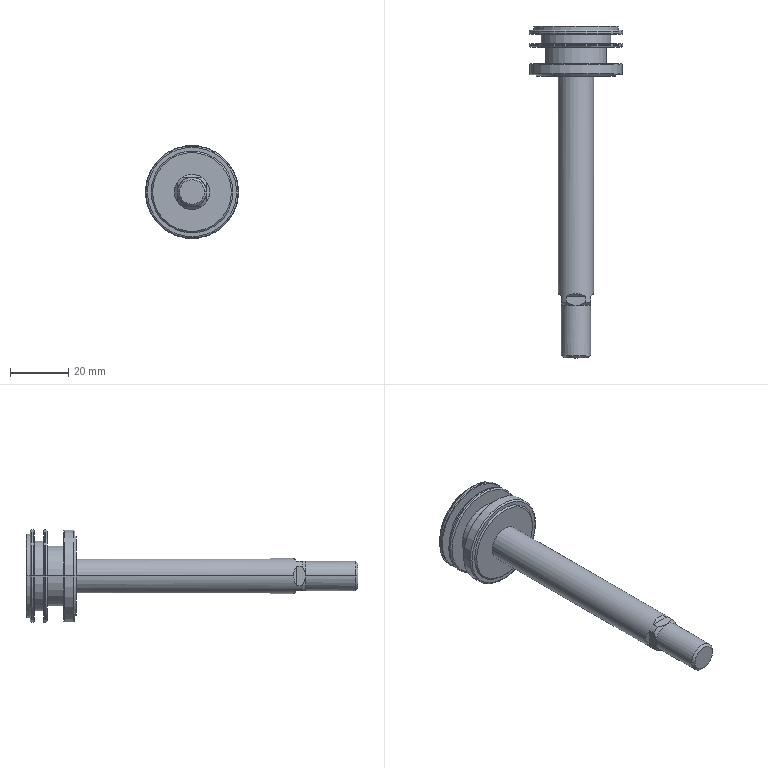Component | SolidWorks | SDAS_32x60_B_0-1_SDAS_32x60_B60_r-1 | 1 solid | 55 faces | box 31.9 x 113.5 x 31.9 mm | volume 19815 mm3 | plane 17 | cylinder 16 | cone 12 | torus 10 | commonest cylinder face diameters 31.9 x4 10 x2 28.9 x2 23.9 x2 20.8 x2 31.6 x2 12 x2
build123d program:
from build123d import *

# Parameters (mm, degrees)
CUT_EXTRUDE1_DEPTH      = 10
CUT_EXTRUDE1_DEPTH_BACK = 10
CUT_EXTRUDE2_DEPTH      = 10
CUT_EXTRUDE2_DEPTH_BACK = 10


with BuildPart() as part:
    # Sketch1 → Revolve1 (revolve)
    with BuildSketch(Plane.XY, mode=Mode.PRIVATE) as revolve1_sk:
        with BuildLine():
            Line((0, 0), (0, 6))
            Line((0, 6), (71.3, 6))
            Line((71.3, 6), (71.3, 13.5))
            Line((71.3, 13.5), (71.8, 14))
            Line((71.8, 14), (71.8, 15.3))
            ThreePointArc((71.8, 15.3), (71.946, 15.654), (72.3, 15.8))
            Line((72.3, 15.8), (75.4, 15.8))
            Line((75.4, 15.8), (75.6, 15.6))
            Line((75.6, 15.6), (75.6, 10.4))
            Line((75.6, 10.4), (81.3, 10.4))
            Line((81.3, 10.4), (81.3, 15.45))
            ThreePointArc((81.3, 15.45), (81.446, 15.804), (81.8, 15.95))
            Line((81.8, 15.95), (82.3, 15.95))
            ThreePointArc((82.3, 15.95), (82.441, 15.891), (82.5, 15.75))
            Line((82.5, 15.75), (82.5, 11.95))
            Line((82.5, 11.95), (85.7, 11.95))
            Line((85.7, 11.95), (85.7, 15.75))
            ThreePointArc((85.7, 15.75), (85.759, 15.891), (85.9, 15.95))
            Line((85.9, 15.95), (86.6, 15.95))
            ThreePointArc((86.6, 15.95), (86.954, 15.804), (87.1, 15.45))
            Line((87.1, 15.45), (87.1, 14.45))
            Line((87.1, 14.45), (88.2, 14.45))
            Line((88.2, 14.45), (88.5, 14.15))
            Line((88.5, 14.15), (88.5, 0))
            Line((88.5, 0), (0, 0))
        make_face()
    revolve(revolve1_sk.sketch.rotate(Axis((88.5, 0, 0), (-1, 0, 0)), 270), axis=Axis((88.5, 0, 0), (-1, 0, 0)))

    # Sketch2 → Revolve2 (revolve)
    with BuildSketch(Plane.XY, mode=Mode.PRIVATE) as revolve2_sk:
        Polygon((-25, 0), (-25, 4.233), (-24.233, 5), (-7, 5), (-6, 6), (0, 6), (0, 0), align=None)
    revolve(revolve2_sk.sketch.rotate(Axis((0, 0, 0), (-1, 0, 0)), 270), axis=Axis((0, 0, 0), (-1, 0, 0)))

    # Sketch3 → Cut-Extrude1 (cut, two sides: drawn at the far end of the back side and taken through both)
    with BuildSketch(Plane(origin=(0, 0, 0), x_dir=(1, 0, 0), z_dir=(0, 1, 0)).offset(-CUT_EXTRUDE1_DEPTH_BACK)):
        Polygon((-35, 25), (-35, -25), (16, -25), (-4, -5), (-7, -5), (-7, -11), (-25, -11), (-25, 11), (-7, 11), (-7, 5), (-4, 5), (16, 25), align=None)
    extrude(amount=CUT_EXTRUDE1_DEPTH + CUT_EXTRUDE1_DEPTH_BACK, mode=Mode.SUBTRACT)

    # Sketch4 → Cut-Extrude2 (cut, two sides: drawn at the far end of the back side and taken through both)
    with BuildSketch(Plane.XY.offset(-CUT_EXTRUDE2_DEPTH_BACK)):
        Polygon((-35, 25), (-35, -25), (16, -25), (-4, -5), (-7, -5), (-7, -11), (-25, -11), (-25, 11), (-7, 11), (-7, 5), (-4, 5), (16, 25), align=None)
    extrude(amount=CUT_EXTRUDE2_DEPTH + CUT_EXTRUDE2_DEPTH_BACK, mode=Mode.SUBTRACT)


solid = part.part

# Placed as in the assembly
solid = solid.moved(Location((174.884, -71.361, 270), (0, 0, 90)))